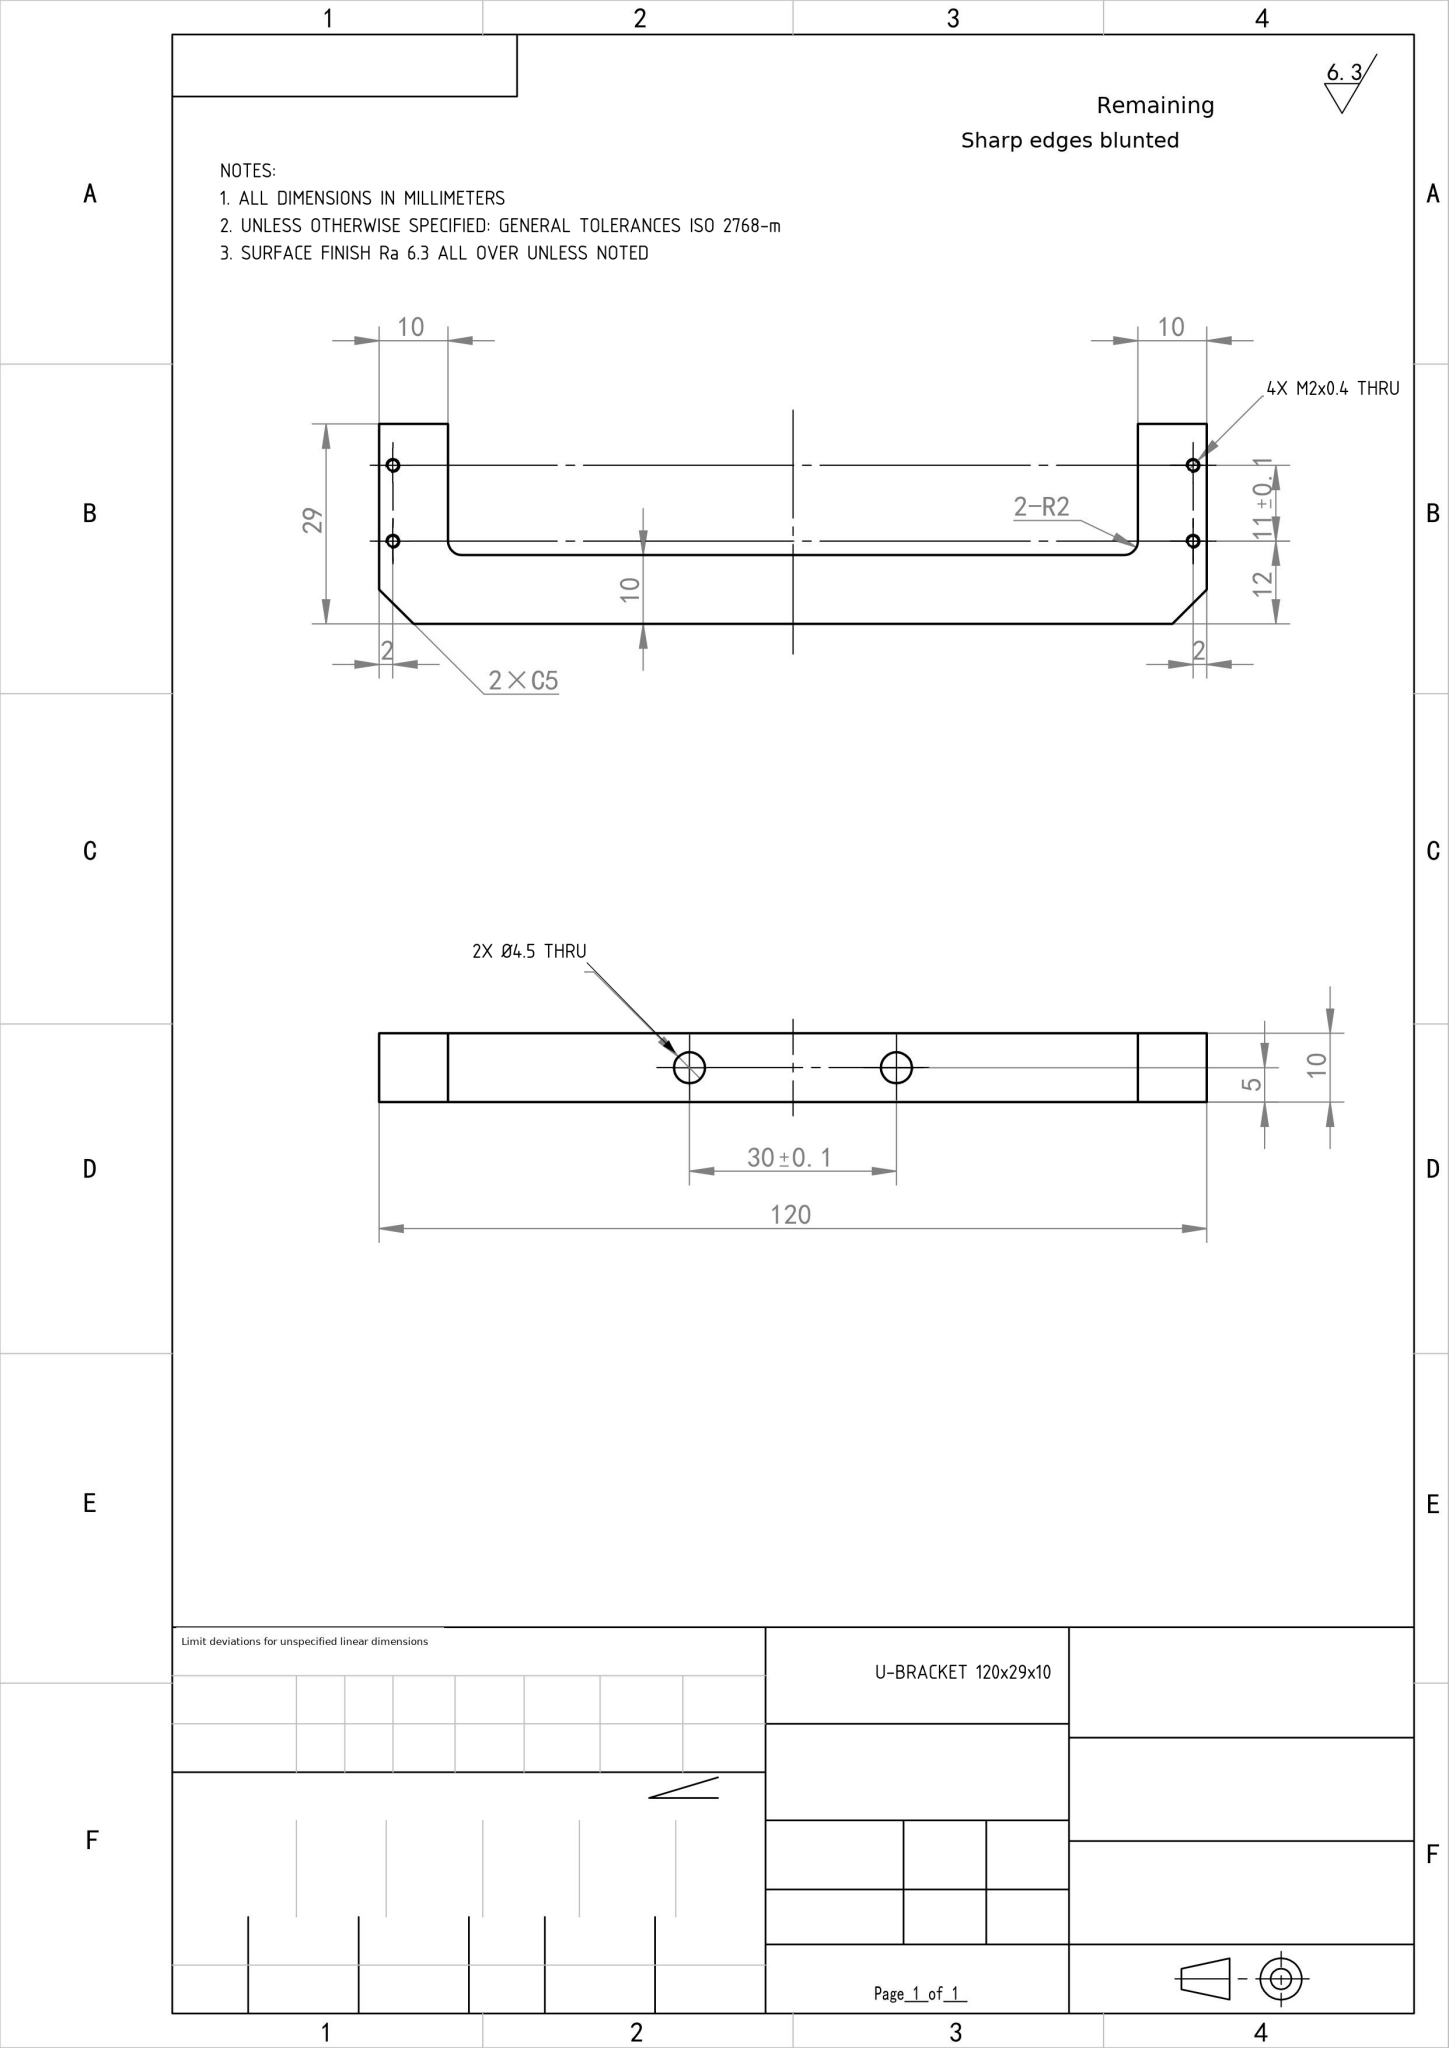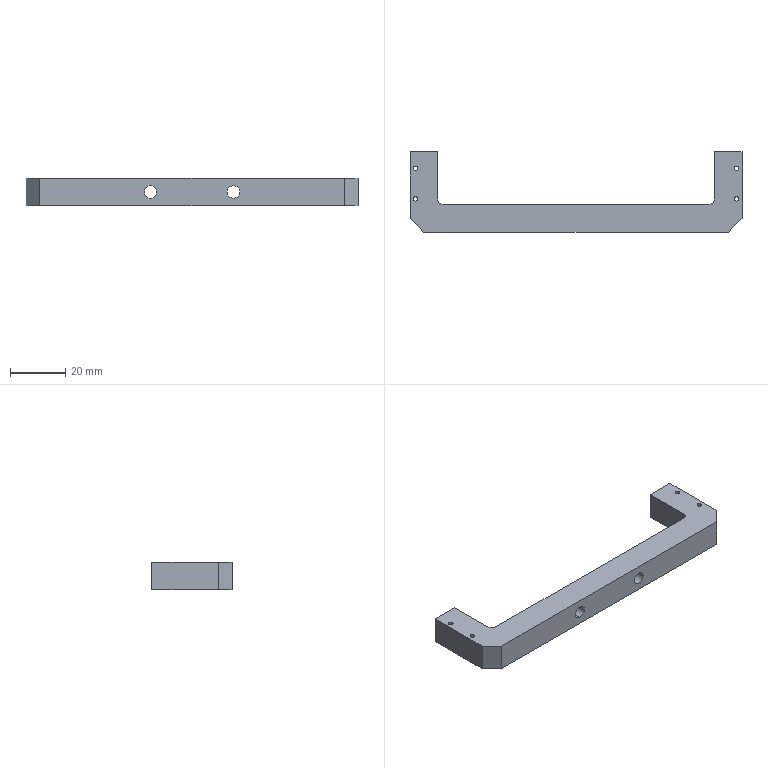Part | NX | mm | 1 solid | 26 faces | box 120 x 29 x 10 mm | volume 15169 mm3 | cylinder 14 | plane 12 | commonest cylinder face diameters 1.6 x8 4.5 x4 4 x2